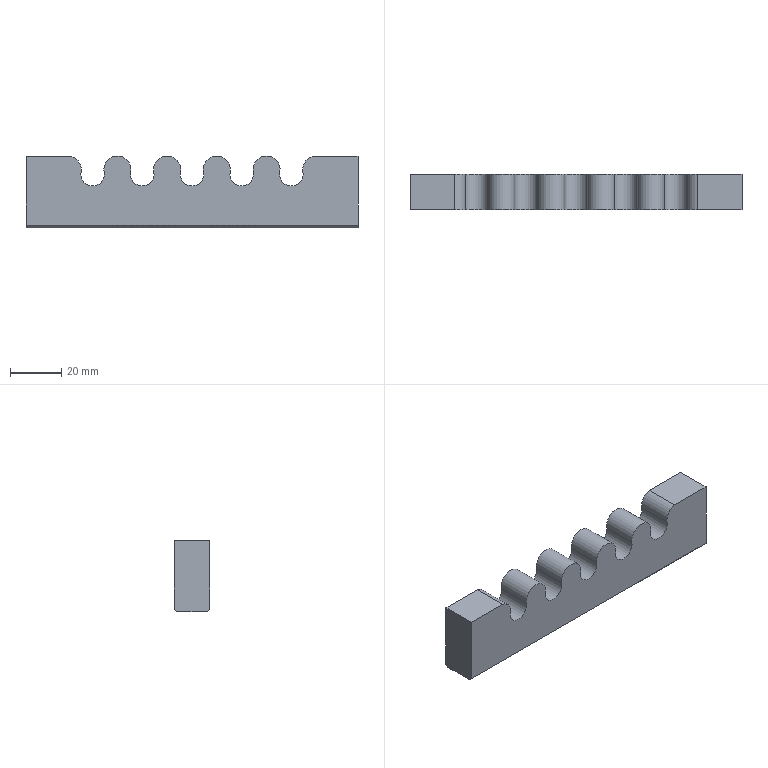Component | NX | 2_RACK | 1 solid | 20 faces | volume 43352 mm3 | cylinder 11 | plane 9 | commonest cylinder face diameters 10.6 x6 9.2 x5